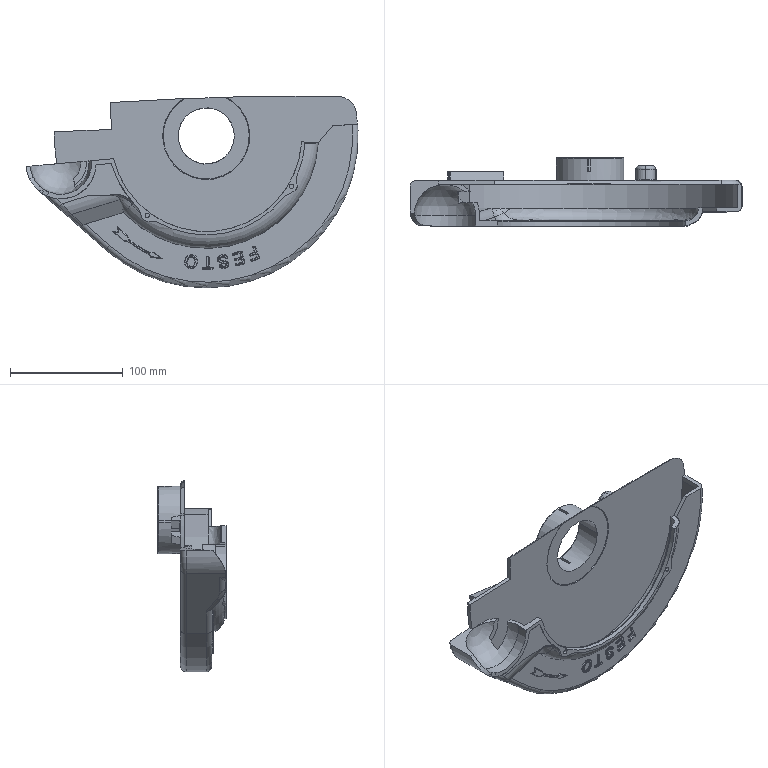Component | SolidWorks | Garde scie int-1 | 1 solid | 375 faces | volume 264114 mm3 | plane 122 | cylinder 121 | spline 62 | torus 57 | cone 10 | sphere 3 | commonest cylinder face diameters 1 x38 2 x32 10 x8 4 x4 270 x3 175.973 x3 40 x3 62 x2